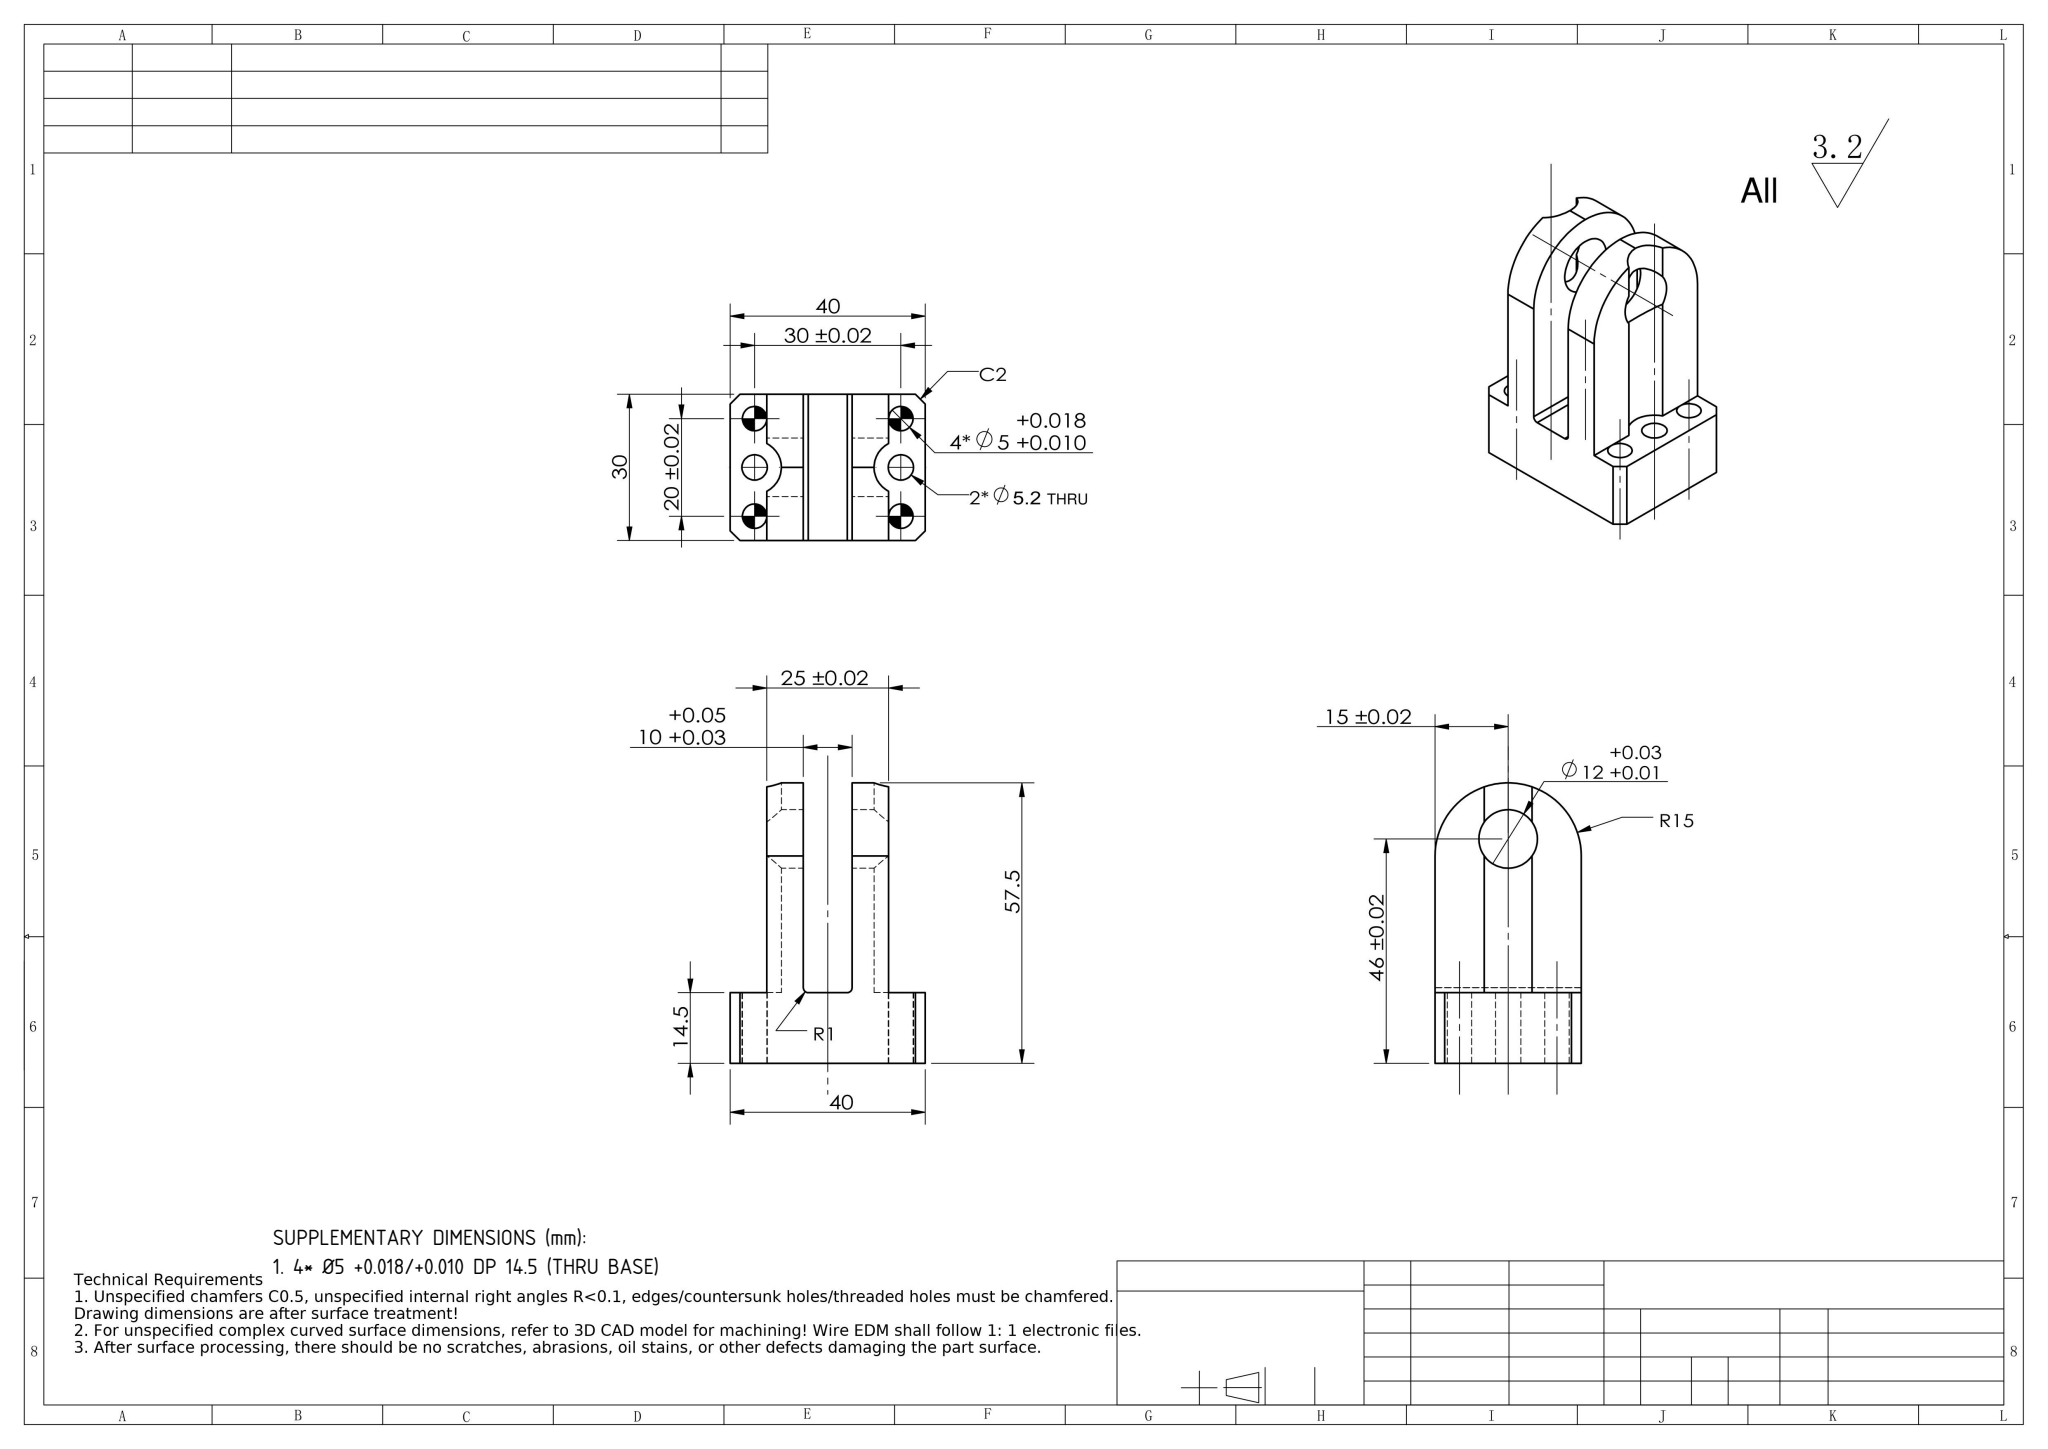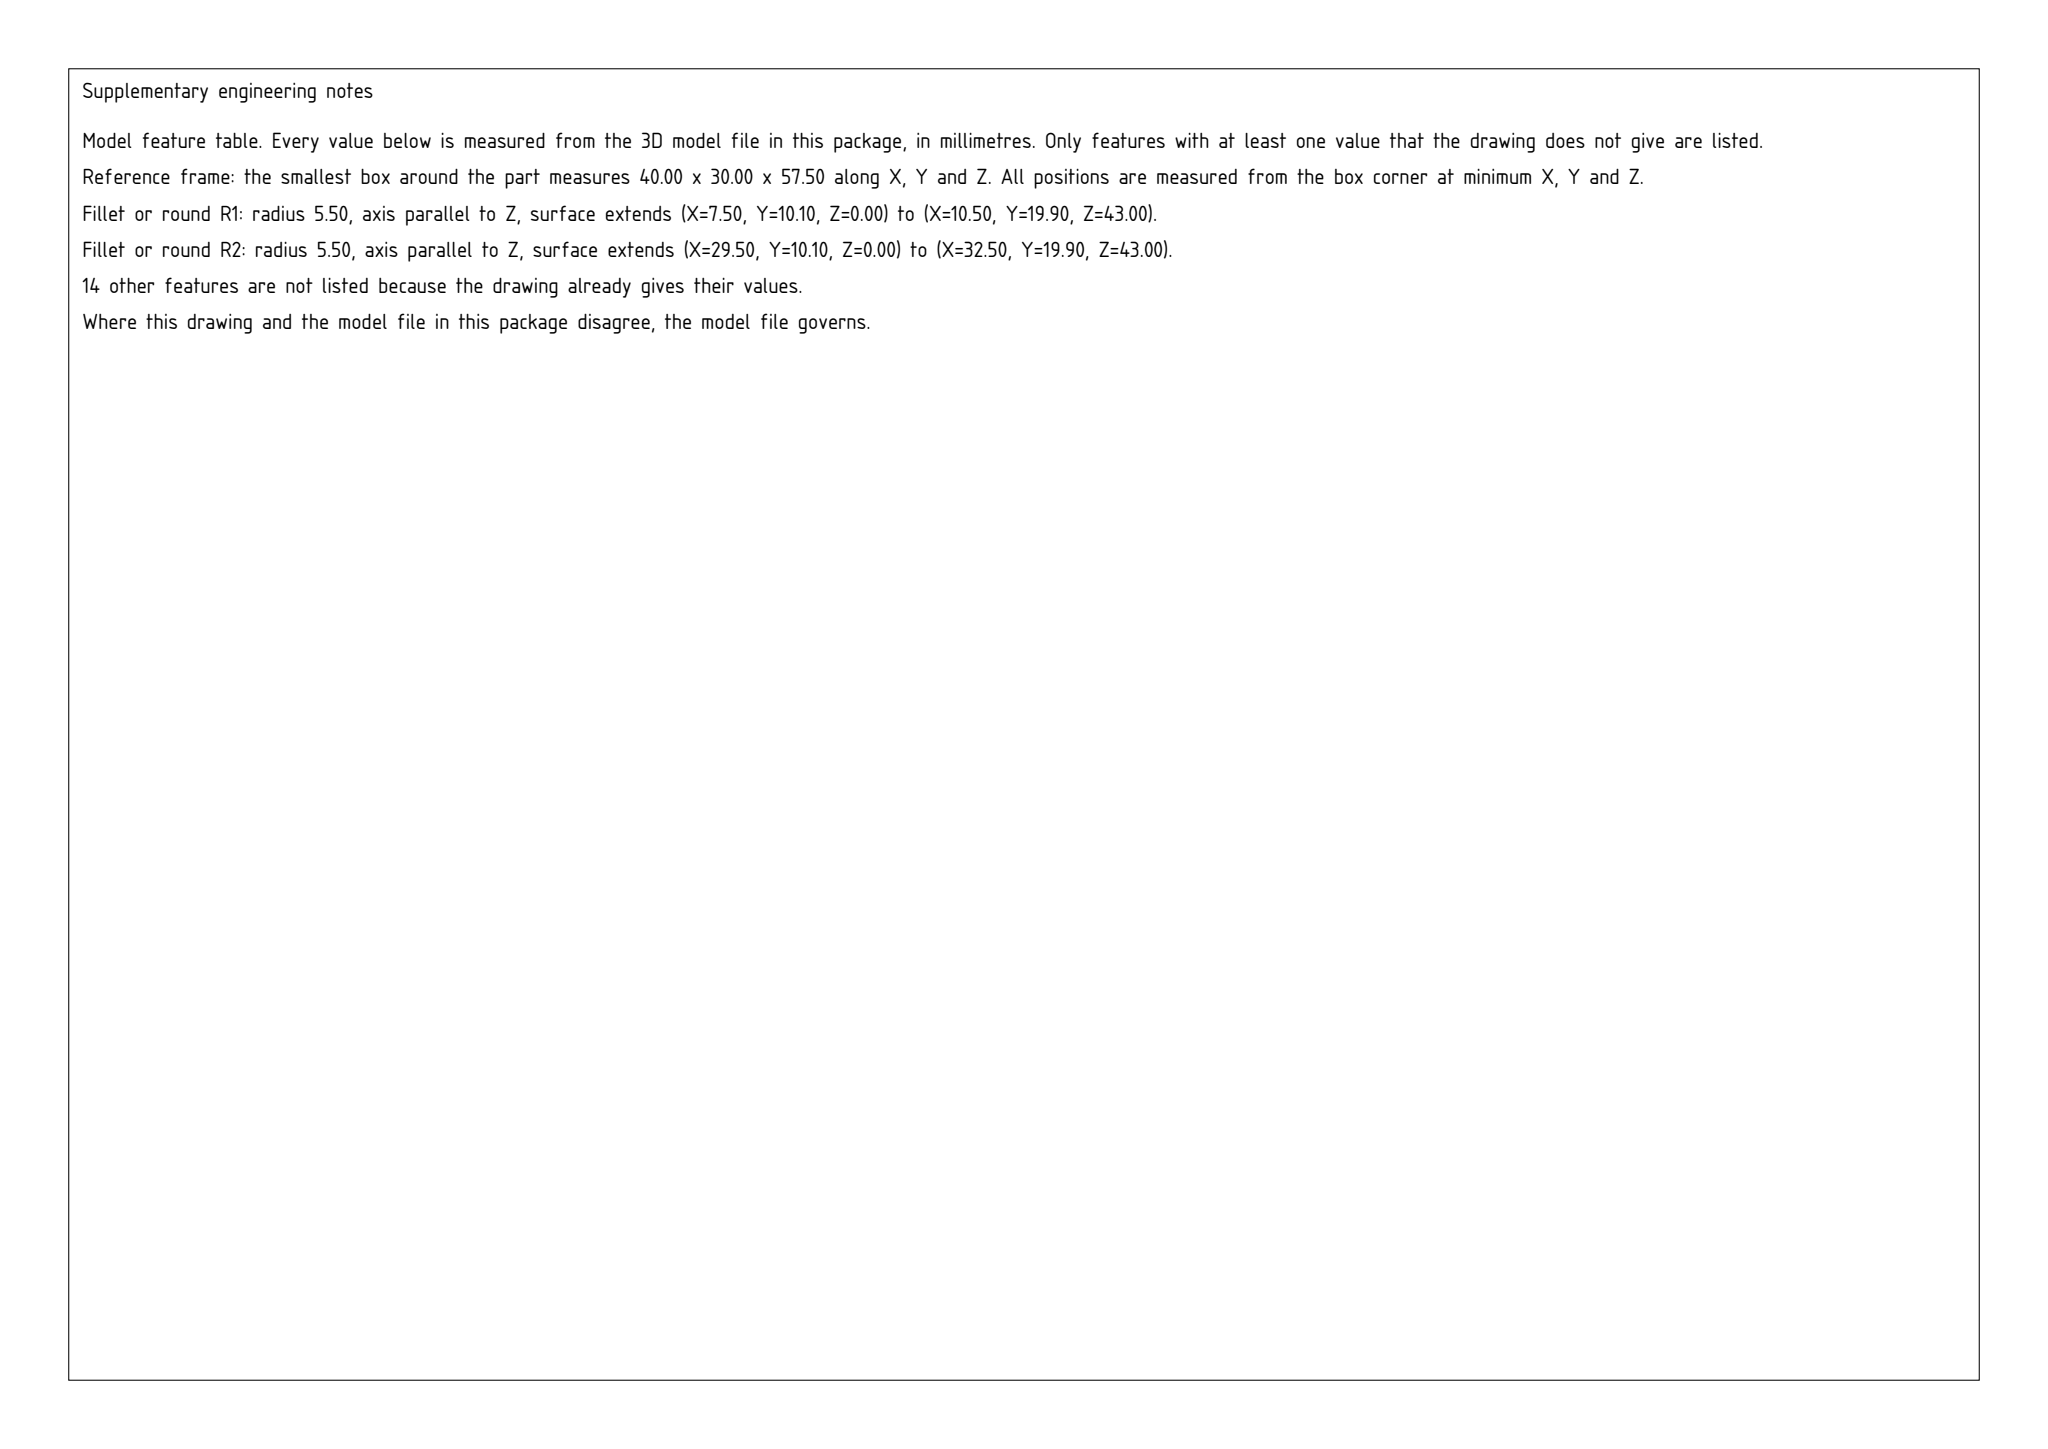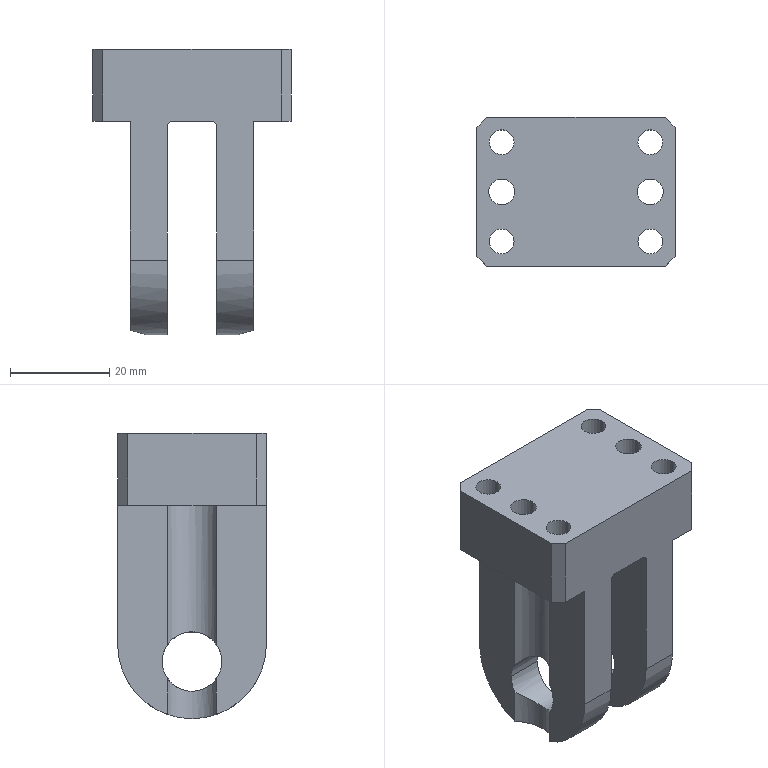Part | SolidWorks | mm | 1 solid | 46 faces | box 40 x 30 x 57.5 mm | volume 30413 mm3 | cylinder 28 | plane 18 | commonest cylinder face diameters 5 x8 11 x6 12 x4 5.2 x4 30 x4 2 x2